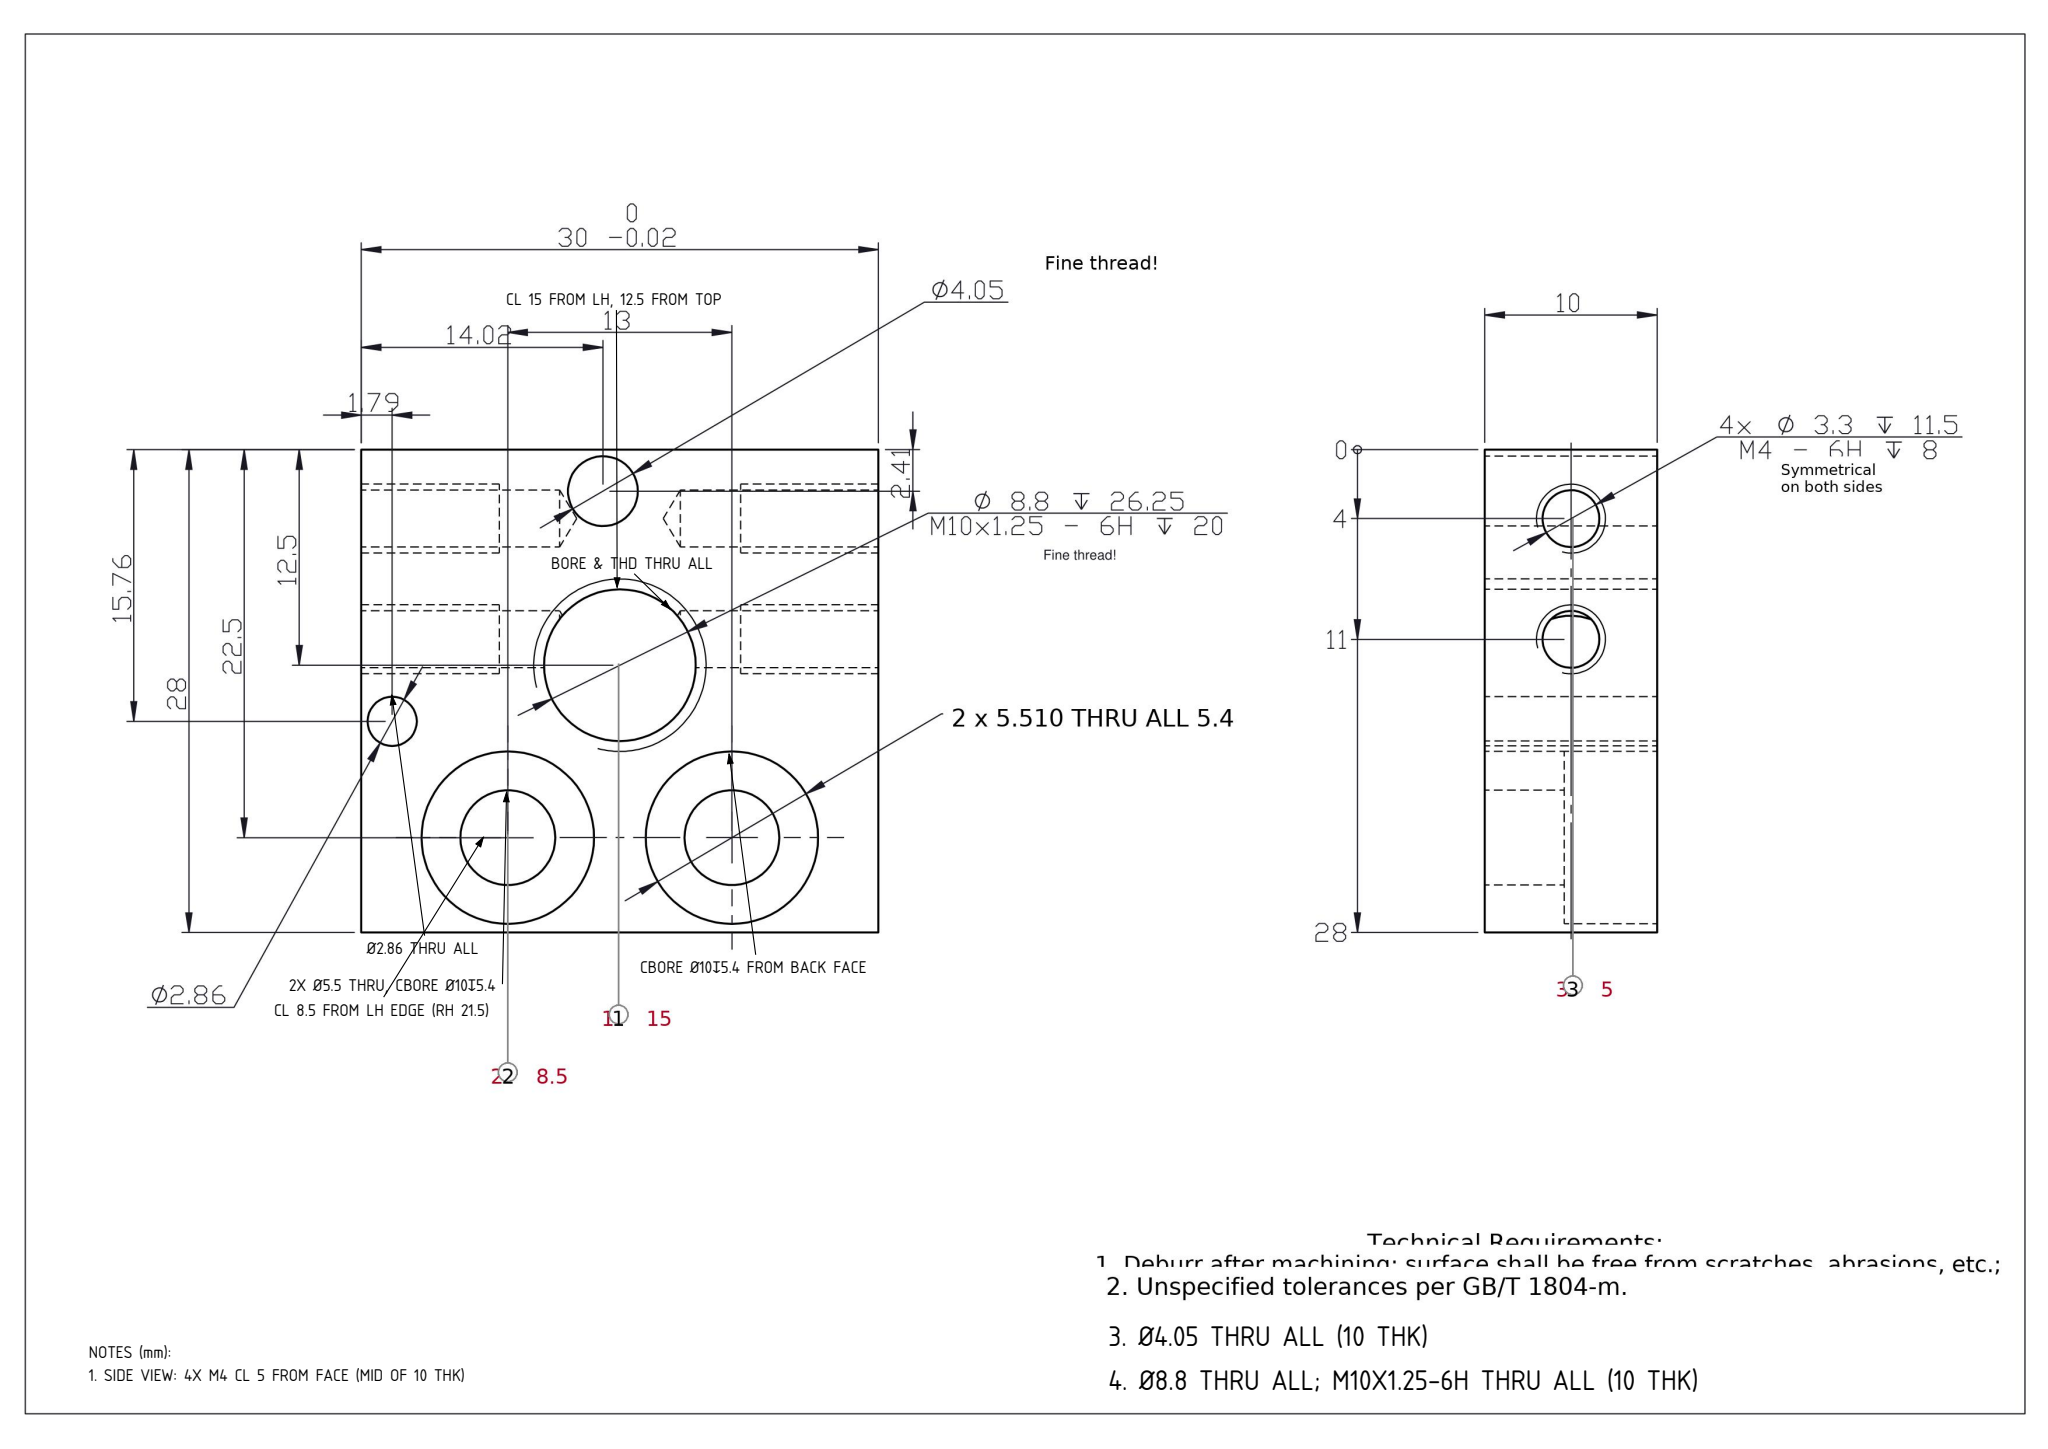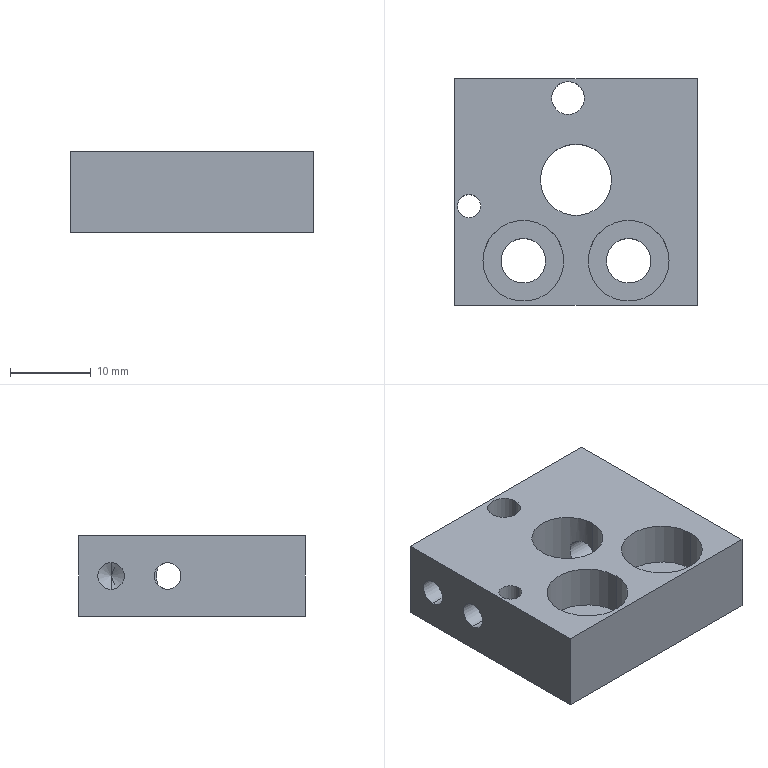Part | SolidWorks | mm | 1 solid | 36 faces | box 30 x 28 x 10 mm | volume 6142 mm3 | cylinder 22 | plane 8 | cone 6 | commonest cylinder face diameters 3.3 x8 10 x4 5.5 x4 4.053 x2 2.855 x2 8.8 x2
Drawing notes:
Ø4.05 THRU ALL (10 THK) | from the solid: hole dia 4.05, axis z at (14.0,25.6), from 0.0 to 10.0 = full 10 thk
Ø2.86 THRU ALL (10 THK) | from the solid: hole dia 2.86, axis z at (1.8,12.2), from 0.0 to 10.0 = full 10 thk
2X Ø5.5 THRU ALL, CBORE Ø10 DP 5.4 FROM BACK FACE | from the solid: Ø5.5 z 0->4.6; Ø10 z 4.6->10.0 (opens at z=10 face); flat z=4.6 cbore bottoms
CBORE Ø10 DP 5.4 MACHINED FROM Z=10 FACE, NOT FRONT FACE | from the solid: Ø10 bores run z 4.6->10.0 at (8.5,5.5) and (21.5,5.5)
Ø8.8 THRU ALL; M10X1.25-6H THRU ALL (10 THK) | from the solid: Ø8.8 bore axis z at (15.0,15.5), from 0.0 to 10.0; plate 10 thk
DISREGARD DP 26.25 / DP 20: BORE + THD ARE THRU ALL (10 THK) | from the solid: bbox_xyz z=10; Ø8.8 bore spans full 0.0-10.0
M10X1.25 BORE CL: 15 FROM LH EDGE, 12.5 FROM TOP EDGE | from the solid: Ø8.8 axis at x=15.0, y=15.5 (28-15.5=12.5 from y=28 edge)
LH Ø5.5 CBORE CL: 8.5 FROM LH EDGE (RH 21.5) | from the solid: Ø5.5/Ø10 axes at x=8.5 and x=21.5, y=5.5
SIDE VIEW: 4X M4 CL 5 FROM FACE (MID OF 10 THK) | from the solid: Ø3.3 x-axis holes at z=5.0, plate 10 thk
build123d program:
from build123d import *

# Parameters (mm, degrees)
SKETCH1_W                                       = 30
SKETCH1_H                                       = 28
BOSS_EXTRUDE1_DEPTH                             = 10
M5_HEX_SOCKET_HEAD_CAP_SCREW_CBORE1_D           = 5.5
M5_HEX_SOCKET_HEAD_CAP_SCREW_CBORE1_CBORE_D     = 10
M5_HEX_SOCKET_HEAD_CAP_SCREW_CBORE1_CBORE_DEPTH = 5.4
M10X1_25_TAPPED_HOLE1_D                         = 8.8
M10X1_25_TAPPED_HOLE1_DEPTH                     = 26.25
M10X1_25_TAPPED_HOLE1_TIP                       = 2.644
M4_TAPPED_HOLE1_D                               = 3.3
M4_TAPPED_HOLE1_DEPTH                           = 11.5
M4_TAPPED_HOLE1_TIP                             = 0.9914
M4_TAPPED_HOLE2_D                               = 3.3
M4_TAPPED_HOLE2_DEPTH                           = 11.5
M4_TAPPED_HOLE2_TIP                             = 0.9914
SKETCH11_R                                      = 2.027
SKETCH11_R_2                                    = 1.428
CUT_EXTRUDE1_DEPTH                              = 10


with BuildPart() as part:
    # Sketch1 → Boss-Extrude1 (new body)
    with BuildSketch(Plane.XY):
        with Locations((15, -14)):
            Rectangle(SKETCH1_W, SKETCH1_H)
    extrude(amount=BOSS_EXTRUDE1_DEPTH)

    # M5 Hex Socket Head Cap Screw CBORE1 (through all)
    with Locations(Plane.XY.offset(10)):
        with Locations((8.5, -22.5), (21.5, -22.5)):
            CounterBoreHole(M5_HEX_SOCKET_HEAD_CAP_SCREW_CBORE1_D / 2, M5_HEX_SOCKET_HEAD_CAP_SCREW_CBORE1_CBORE_D / 2, M5_HEX_SOCKET_HEAD_CAP_SCREW_CBORE1_CBORE_DEPTH)

    # M10x1.25 Tapped Hole1
    with Locations(Plane.XY.offset(10)):
        with Locations((15, -12.5)):
            Hole(M10X1_25_TAPPED_HOLE1_D / 2, depth=M10X1_25_TAPPED_HOLE1_DEPTH)
            with Locations((0, 0, -(M10X1_25_TAPPED_HOLE1_DEPTH + M10X1_25_TAPPED_HOLE1_TIP / 2))):  # 118° drill point
                Cone(0, M10X1_25_TAPPED_HOLE1_D / 2, M10X1_25_TAPPED_HOLE1_TIP, mode=Mode.SUBTRACT)

    # M4 Tapped Hole1
    with Locations(Plane.ZY):
        with Locations((5, -4), (5, -11)):
            Hole(M4_TAPPED_HOLE1_D / 2, depth=M4_TAPPED_HOLE1_DEPTH)
            with Locations((0, 0, -(M4_TAPPED_HOLE1_DEPTH + M4_TAPPED_HOLE1_TIP / 2))):  # 118° drill point
                Cone(0, M4_TAPPED_HOLE1_D / 2, M4_TAPPED_HOLE1_TIP, mode=Mode.SUBTRACT)

    # M4 Tapped Hole2
    with Locations(Plane(origin=(30, 0, 0), x_dir=(0, 0, -1), z_dir=(1, 0, 0))):
        with Locations((-5, -4), (-5, -11)):
            Hole(M4_TAPPED_HOLE2_D / 2, depth=M4_TAPPED_HOLE2_DEPTH)
            with Locations((0, 0, -(M4_TAPPED_HOLE2_DEPTH + M4_TAPPED_HOLE2_TIP / 2))):  # 118° drill point
                Cone(0, M4_TAPPED_HOLE2_D / 2, M4_TAPPED_HOLE2_TIP, mode=Mode.SUBTRACT)

    # Sketch11 → Cut-Extrude1 (cut)
    with BuildSketch(Plane.XY.offset(10)):
        with Locations((14.016, -2.407)):
            Circle(SKETCH11_R)
        with Locations((1.792, -15.755)):
            Circle(SKETCH11_R_2)
    extrude(amount=-CUT_EXTRUDE1_DEPTH, mode=Mode.SUBTRACT)


solid = part.part